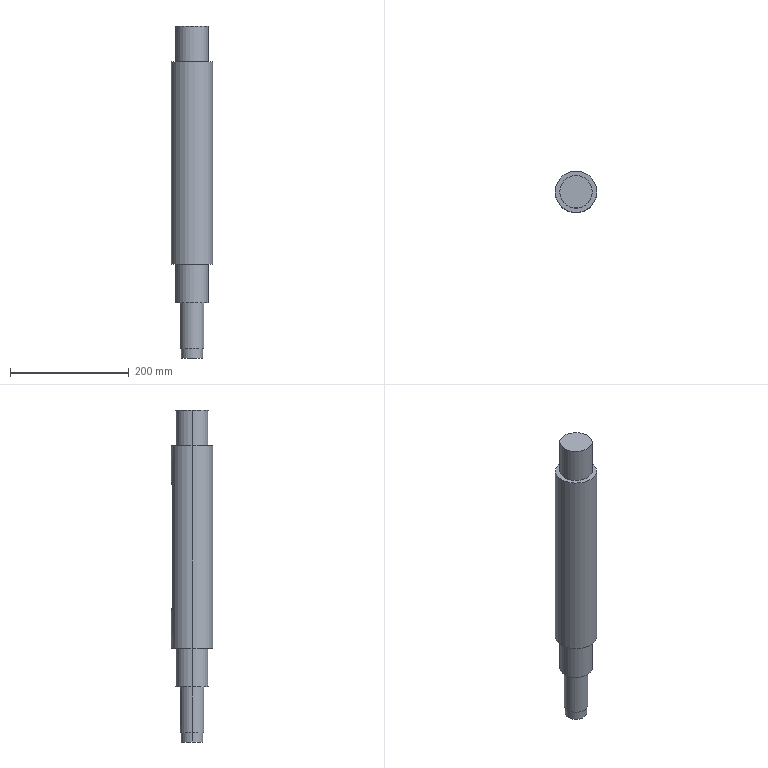Component | SolidWorks | Spindle-1 | 1 solid | 26 faces | box 70 x 70 x 560 mm | volume 1692469 mm3 | cylinder 14 | plane 12 | commonest cylinder face diameters 55 x4 70 x2 40 x2 36 x2 20 x2 12 x2
STEP:
#1=COLOUR_RGB('',0.7922,0.8196,0.9333);
#2=FILL_AREA_STYLE_COLOUR('',#1);
#3=FILL_AREA_STYLE('',(#2));
#4=SURFACE_STYLE_FILL_AREA(#3);
#5=SURFACE_SIDE_STYLE('',(#4));
#6=SURFACE_STYLE_USAGE(.BOTH.,#5);
#7=PRESENTATION_STYLE_ASSIGNMENT((#6));
#8=CARTESIAN_POINT('',(8.661,10.159,-3.886));
#9=VERTEX_POINT('',#8);
#10=CARTESIAN_POINT('',(8.661,10.159,3.988));
#11=VERTEX_POINT('',#10);
#12=CARTESIAN_POINT('',(8.661,10.159,9.106));
#13=DIRECTION('',(0.,0.,1.));
#14=VECTOR('',#13,39.37);
#15=LINE('',#12,#14);
#16=EDGE_CURVE('',#9,#11,#15,.T.);
#17=ORIENTED_EDGE('',*,*,#16,.T.);
#18=CARTESIAN_POINT('',(7.874,10.159,3.988));
#19=VERTEX_POINT('',#18);
#20=CARTESIAN_POINT('',(8.661,10.159,3.988));
#21=CARTESIAN_POINT('',(8.661,10.159,4.014));
#22=CARTESIAN_POINT('',(8.659,10.16,4.04));
#23=CARTESIAN_POINT('',(8.651,10.162,4.078));
#24=CARTESIAN_POINT('',(8.648,10.163,4.09));
#25=CARTESIAN_POINT('',(8.641,10.165,4.115));
#26=CARTESIAN_POINT('',(8.636,10.166,4.127));
#27=CARTESIAN_POINT('',(8.621,10.17,4.163));
#28=CARTESIAN_POINT('',(8.609,10.174,4.186));
#29=CARTESIAN_POINT('',(8.588,10.179,4.218));
#30=CARTESIAN_POINT('',(8.58,10.181,4.228));
#31=CARTESIAN_POINT('',(8.564,10.184,4.248));
#32=CARTESIAN_POINT('',(8.555,10.186,4.258));
#33=CARTESIAN_POINT('',(8.528,10.192,4.285));
#34=CARTESIAN_POINT('',(8.508,10.196,4.301));
#35=CARTESIAN_POINT('',(8.465,10.202,4.33));
#36=CARTESIAN_POINT('',(8.443,10.206,4.342));
#37=CARTESIAN_POINT('',(8.407,10.21,4.357));
#38=CARTESIAN_POINT('',(8.395,10.211,4.361));
#39=CARTESIAN_POINT('',(8.37,10.213,4.368));
#40=CARTESIAN_POINT('',(8.358,10.214,4.372));
#41=CARTESIAN_POINT('',(8.32,10.216,4.379));
#42=CARTESIAN_POINT('',(8.294,10.217,4.382));
#43=CARTESIAN_POINT('',(8.242,10.217,4.382));
#44=CARTESIAN_POINT('',(8.216,10.216,4.379));
#45=CARTESIAN_POINT('',(8.165,10.213,4.369));
#46=CARTESIAN_POINT('',(8.141,10.211,4.362));
#47=CARTESIAN_POINT('',(8.105,10.207,4.347));
#48=CARTESIAN_POINT('',(8.093,10.205,4.341));
#49=CARTESIAN_POINT('',(8.07,10.202,4.329));
#50=CARTESIAN_POINT('',(8.06,10.201,4.323));
#51=CARTESIAN_POINT('',(8.038,10.197,4.308));
#52=CARTESIAN_POINT('',(8.028,10.196,4.301));
#53=CARTESIAN_POINT('',(8.008,10.192,4.284));
#54=CARTESIAN_POINT('',(7.999,10.19,4.276));
#55=CARTESIAN_POINT('',(7.971,10.184,4.248));
#56=CARTESIAN_POINT('',(7.955,10.181,4.229));
#57=CARTESIAN_POINT('',(7.927,10.174,4.186));
#58=CARTESIAN_POINT('',(7.914,10.17,4.163));
#59=CARTESIAN_POINT('',(7.894,10.165,4.116));
#60=CARTESIAN_POINT('',(7.887,10.163,4.091));
#61=CARTESIAN_POINT('',(7.879,10.161,4.053));
#62=CARTESIAN_POINT('',(7.877,10.16,4.04));
#63=CARTESIAN_POINT('',(7.875,10.159,4.014));
#64=CARTESIAN_POINT('',(7.874,10.159,4.001));
#65=CARTESIAN_POINT('',(7.874,10.159,3.988));
#66=B_SPLINE_CURVE_WITH_KNOTS('',3,(#20,#21,#22,#23,#24,#25,#26,#27,#28,#29,#30,#31,#32,#33,#34,#35,#36,#37,#38,#39,#40,#41,#42,#43,#44,#45,#46,#47,#48,#49,#50,#51,#52,#53,#54,#55,#56,#57,#58,#59,#60,#61,#62,#63,#64,#65),.UNSPECIFIED.,.F.,.F.,(4,2,2,2,2,2,2,2,2,2,2,2,2,2,2,2,2,2,2,2,2,2,4),(0.,0.001964,0.002945,0.003927,0.005891,0.006873,0.007855,0.009818,0.01178,0.01276,0.01375,0.01571,0.01767,0.01964,0.02062,0.0216,0.02258,0.02356,0.02553,0.02749,0.02945,0.03044,0.03142),.UNSPECIFIED.);
#67=EDGE_CURVE('',#11,#19,#66,.T.);
#68=ORIENTED_EDGE('',*,*,#67,.T.);
#69=CARTESIAN_POINT('',(7.874,10.159,-3.886));
#70=VERTEX_POINT('',#69);
#71=CARTESIAN_POINT('',(7.874,10.159,9.106));
#72=DIRECTION('',(0.,0.,-1.));
#73=VECTOR('',#72,39.37);
#74=LINE('',#71,#73);
#75=EDGE_CURVE('',#19,#70,#74,.T.);
#76=ORIENTED_EDGE('',*,*,#75,.T.);
#77=CARTESIAN_POINT('',(7.874,10.159,-3.886));
#78=CARTESIAN_POINT('',(7.874,10.159,-3.912));
#79=CARTESIAN_POINT('',(7.877,10.16,-3.938));
#80=CARTESIAN_POINT('',(7.884,10.162,-3.976));
#81=CARTESIAN_POINT('',(7.887,10.163,-3.988));
#82=CARTESIAN_POINT('',(7.895,10.165,-4.013));
#83=CARTESIAN_POINT('',(7.899,10.166,-4.025));
#84=CARTESIAN_POINT('',(7.914,10.17,-4.061));
#85=CARTESIAN_POINT('',(7.926,10.174,-4.083));
#86=CARTESIAN_POINT('',(7.948,10.179,-4.115));
#87=CARTESIAN_POINT('',(7.955,10.181,-4.126));
#88=CARTESIAN_POINT('',(7.972,10.184,-4.146));
#89=CARTESIAN_POINT('',(7.98,10.186,-4.155));
#90=CARTESIAN_POINT('',(8.007,10.192,-4.182));
#91=CARTESIAN_POINT('',(8.027,10.196,-4.199));
#92=CARTESIAN_POINT('',(8.07,10.202,-4.227));
#93=CARTESIAN_POINT('',(8.093,10.206,-4.239));
#94=CARTESIAN_POINT('',(8.128,10.21,-4.254));
#95=CARTESIAN_POINT('',(8.14,10.211,-4.259));
#96=CARTESIAN_POINT('',(8.165,10.213,-4.266));
#97=CARTESIAN_POINT('',(8.178,10.214,-4.269));
#98=CARTESIAN_POINT('',(8.216,10.216,-4.277));
#99=CARTESIAN_POINT('',(8.242,10.217,-4.28));
#100=CARTESIAN_POINT('',(8.293,10.217,-4.28));
#101=CARTESIAN_POINT('',(8.319,10.216,-4.277));
#102=CARTESIAN_POINT('',(8.37,10.213,-4.267));
#103=CARTESIAN_POINT('',(8.395,10.211,-4.259));
#104=CARTESIAN_POINT('',(8.43,10.207,-4.245));
#105=CARTESIAN_POINT('',(8.442,10.205,-4.239));
#106=CARTESIAN_POINT('',(8.465,10.202,-4.227));
#107=CARTESIAN_POINT('',(8.476,10.201,-4.22));
#108=CARTESIAN_POINT('',(8.497,10.197,-4.206));
#109=CARTESIAN_POINT('',(8.507,10.196,-4.198));
#110=CARTESIAN_POINT('',(8.527,10.192,-4.182));
#111=CARTESIAN_POINT('',(8.537,10.19,-4.173));
#112=CARTESIAN_POINT('',(8.564,10.184,-4.146));
#113=CARTESIAN_POINT('',(8.58,10.181,-4.126));
#114=CARTESIAN_POINT('',(8.609,10.174,-4.084));
#115=CARTESIAN_POINT('',(8.621,10.17,-4.061));
#116=CARTESIAN_POINT('',(8.641,10.165,-4.013));
#117=CARTESIAN_POINT('',(8.649,10.163,-3.989));
#118=CARTESIAN_POINT('',(8.656,10.161,-3.951));
#119=CARTESIAN_POINT('',(8.658,10.16,-3.938));
#120=CARTESIAN_POINT('',(8.661,10.159,-3.912));
#121=CARTESIAN_POINT('',(8.661,10.159,-3.899));
#122=CARTESIAN_POINT('',(8.661,10.159,-3.886));
#123=B_SPLINE_CURVE_WITH_KNOTS('',3,(#77,#78,#79,#80,#81,#82,#83,#84,#85,#86,#87,#88,#89,#90,#91,#92,#93,#94,#95,#96,#97,#98,#99,#100,#101,#102,#103,#104,#105,#106,#107,#108,#109,#110,#111,#112,#113,#114,#115,#116,#117,#118,#119,#120,#121,#122),.UNSPECIFIED.,.F.,.F.,(4,2,2,2,2,2,2,2,2,2,2,2,2,2,2,2,2,2,2,2,2,2,4),(0.,0.001964,0.002945,0.003927,0.005891,0.006873,0.007855,0.009818,0.01178,0.01276,0.01375,0.01571,0.01767,0.01964,0.02062,0.0216,0.02258,0.02356,0.02553,0.02749,0.02945,0.03044,0.03142),.UNSPECIFIED.);
#124=EDGE_CURVE('',#70,#9,#123,.T.);
#125=ORIENTED_EDGE('',*,*,#124,.T.);
#126=EDGE_LOOP('',(#17,#68,#76,#125));
#127=FACE_BOUND('',#126,.T.);
#128=CARTESIAN_POINT('',(9.646,8.839,-6.72));
#129=VERTEX_POINT('',#128);
#130=CARTESIAN_POINT('',(6.89,8.839,-6.72));
#131=VERTEX_POINT('',#130);
#132=CARTESIAN_POINT('',(8.268,8.839,-6.72));
#133=DIRECTION('',(0.,0.,1.));
#134=DIRECTION('',(1.,0.,0.));
#135=AXIS2_PLACEMENT_3D('',#132,#133,#134);
#136=CIRCLE('',#135,1.378);
#137=EDGE_CURVE('',#129,#131,#136,.T.);
#138=ORIENTED_EDGE('',*,*,#137,.T.);
#139=CARTESIAN_POINT('',(6.89,8.839,6.744));
#140=VERTEX_POINT('',#139);
#141=CARTESIAN_POINT('',(6.89,8.839,9.106));
#142=DIRECTION('',(0.,0.,1.));
#143=VECTOR('',#142,39.37);
#144=LINE('',#141,#143);
#145=EDGE_CURVE('',#131,#140,#144,.T.);
#146=ORIENTED_EDGE('',*,*,#145,.T.);
#147=CARTESIAN_POINT('',(9.646,8.839,6.744));
#148=VERTEX_POINT('',#147);
#149=CARTESIAN_POINT('',(8.268,8.839,6.744));
#150=DIRECTION('',(0.,0.,-1.));
#151=DIRECTION('',(1.,0.,0.));
#152=AXIS2_PLACEMENT_3D('',#149,#150,#151);
#153=CIRCLE('',#152,1.378);
#154=EDGE_CURVE('',#140,#148,#153,.T.);
#155=ORIENTED_EDGE('',*,*,#154,.T.);
#156=CARTESIAN_POINT('',(9.646,8.839,9.106));
#157=DIRECTION('',(0.,0.,1.));
#158=VECTOR('',#157,39.37);
#159=LINE('',#156,#158);
#160=EDGE_CURVE('',#129,#148,#159,.T.);
#161=ORIENTED_EDGE('',*,*,#160,.F.);
#162=EDGE_LOOP('',(#138,#146,#155,#161));
#163=FACE_OUTER_BOUND('',#162,.T.);
#164=CARTESIAN_POINT('',(8.268,8.839,9.106));
#165=DIRECTION('',(0.,0.,1.));
#166=DIRECTION('',(1.,0.,0.));
#167=AXIS2_PLACEMENT_3D('',#164,#165,#166);
#168=CYLINDRICAL_SURFACE('',#167,1.378);
#169=ADVANCED_FACE('',(#127,#163),#168,.T.);
#170=CARTESIAN_POINT('',(9.35,8.839,6.744));
#171=VERTEX_POINT('',#170);
#172=CARTESIAN_POINT('',(7.185,8.839,6.744));
#173=VERTEX_POINT('',#172);
#174=CARTESIAN_POINT('',(8.268,8.839,6.744));
#175=DIRECTION('',(0.,0.,1.));
#176=DIRECTION('',(1.,0.,0.));
#177=AXIS2_PLACEMENT_3D('',#174,#175,#176);
#178=CIRCLE('',#177,1.083);
#179=EDGE_CURVE('',#171,#173,#178,.T.);
#180=ORIENTED_EDGE('',*,*,#179,.T.);
#181=CARTESIAN_POINT('',(7.185,8.839,9.106));
#182=VERTEX_POINT('',#181);
#183=CARTESIAN_POINT('',(7.185,8.839,9.106));
#184=DIRECTION('',(0.,0.,1.));
#185=VECTOR('',#184,39.37);
#186=LINE('',#183,#185);
#187=EDGE_CURVE('',#173,#182,#186,.T.);
#188=ORIENTED_EDGE('',*,*,#187,.T.);
#189=CARTESIAN_POINT('',(9.35,8.839,9.106));
#190=VERTEX_POINT('',#189);
#191=CARTESIAN_POINT('',(8.268,8.839,9.106));
#192=DIRECTION('',(0.,0.,-1.));
#193=DIRECTION('',(1.,0.,0.));
#194=AXIS2_PLACEMENT_3D('',#191,#192,#193);
#195=CIRCLE('',#194,1.083);
#196=EDGE_CURVE('',#182,#190,#195,.T.);
#197=ORIENTED_EDGE('',*,*,#196,.T.);
#198=CARTESIAN_POINT('',(9.35,8.839,9.106));
#199=DIRECTION('',(0.,0.,1.));
#200=VECTOR('',#199,39.37);
#201=LINE('',#198,#200);
#202=EDGE_CURVE('',#171,#190,#201,.T.);
#203=ORIENTED_EDGE('',*,*,#202,.F.);
#204=EDGE_LOOP('',(#180,#188,#197,#203));
#205=FACE_OUTER_BOUND('',#204,.T.);
#206=CARTESIAN_POINT('',(8.268,8.839,9.106));
#207=DIRECTION('',(0.,0.,1.));
#208=DIRECTION('',(1.,0.,0.));
#209=AXIS2_PLACEMENT_3D('',#206,#207,#208);
#210=CYLINDRICAL_SURFACE('',#209,1.083);
#211=ADVANCED_FACE('',(#205),#210,.T.);
#212=CARTESIAN_POINT('',(9.35,8.839,-9.28));
#213=VERTEX_POINT('',#212);
#214=CARTESIAN_POINT('',(7.185,8.839,-9.28));
#215=VERTEX_POINT('',#214);
#216=CARTESIAN_POINT('',(8.268,8.839,-9.28));
#217=DIRECTION('',(0.,0.,1.));
#218=DIRECTION('',(1.,0.,0.));
#219=AXIS2_PLACEMENT_3D('',#216,#217,#218);
#220=CIRCLE('',#219,1.083);
#221=EDGE_CURVE('',#213,#215,#220,.T.);
#222=ORIENTED_EDGE('',*,*,#221,.T.);
#223=CARTESIAN_POINT('',(7.185,8.839,-6.72));
#224=VERTEX_POINT('',#223);
#225=CARTESIAN_POINT('',(7.185,8.839,9.106));
#226=DIRECTION('',(0.,0.,1.));
#227=VECTOR('',#226,39.37);
#228=LINE('',#225,#227);
#229=EDGE_CURVE('',#215,#224,#228,.T.);
#230=ORIENTED_EDGE('',*,*,#229,.T.);
#231=CARTESIAN_POINT('',(9.35,8.839,-6.72));
#232=VERTEX_POINT('',#231);
#233=CARTESIAN_POINT('',(8.268,8.839,-6.72));
#234=DIRECTION('',(0.,0.,-1.));
#235=DIRECTION('',(1.,0.,0.));
#236=AXIS2_PLACEMENT_3D('',#233,#234,#235);
#237=CIRCLE('',#236,1.083);
#238=EDGE_CURVE('',#224,#232,#237,.T.);
#239=ORIENTED_EDGE('',*,*,#238,.T.);
#240=CARTESIAN_POINT('',(9.35,8.839,9.106));
#241=DIRECTION('',(0.,0.,1.));
#242=VECTOR('',#241,39.37);
#243=LINE('',#240,#242);
#244=EDGE_CURVE('',#213,#232,#243,.T.);
#245=ORIENTED_EDGE('',*,*,#244,.F.);
#246=EDGE_LOOP('',(#222,#230,#239,#245));
#247=FACE_OUTER_BOUND('',#246,.T.);
#248=CARTESIAN_POINT('',(8.268,8.839,9.106));
#249=DIRECTION('',(0.,0.,1.));
#250=DIRECTION('',(1.,0.,0.));
#251=AXIS2_PLACEMENT_3D('',#248,#249,#250);
#252=CYLINDRICAL_SURFACE('',#251,1.083);
#253=ADVANCED_FACE('',(#247),#252,.T.);
#254=CARTESIAN_POINT('',(8.504,9.59,-11.72));
#255=VERTEX_POINT('',#254);
#256=CARTESIAN_POINT('',(8.504,9.59,-9.713));
#257=VERTEX_POINT('',#256);
#258=CARTESIAN_POINT('',(8.504,9.59,9.106));
#259=DIRECTION('',(0.,0.,1.));
#260=VECTOR('',#259,39.37);
#261=LINE('',#258,#260);
#262=EDGE_CURVE('',#255,#257,#261,.T.);
#263=ORIENTED_EDGE('',*,*,#262,.T.);
#264=CARTESIAN_POINT('',(8.031,9.59,-9.713));
#265=VERTEX_POINT('',#264);
#266=CARTESIAN_POINT('',(8.504,9.59,-9.713));
#267=CARTESIAN_POINT('',(8.504,9.59,-9.697));
#268=CARTESIAN_POINT('',(8.502,9.59,-9.681));
#269=CARTESIAN_POINT('',(8.498,9.592,-9.659));
#270=CARTESIAN_POINT('',(8.496,9.592,-9.651));
#271=CARTESIAN_POINT('',(8.491,9.594,-9.636));
#272=CARTESIAN_POINT('',(8.489,9.594,-9.629));
#273=CARTESIAN_POINT('',(8.48,9.597,-9.608));
#274=CARTESIAN_POINT('',(8.473,9.599,-9.594));
#275=CARTESIAN_POINT('',(8.46,9.602,-9.575));
#276=CARTESIAN_POINT('',(8.455,9.603,-9.569));
#277=CARTESIAN_POINT('',(8.445,9.606,-9.557));
#278=CARTESIAN_POINT('',(8.44,9.607,-9.551));
#279=CARTESIAN_POINT('',(8.424,9.61,-9.535));
#280=CARTESIAN_POINT('',(8.412,9.613,-9.525));
#281=CARTESIAN_POINT('',(8.386,9.617,-9.508));
#282=CARTESIAN_POINT('',(8.373,9.619,-9.5));
#283=CARTESIAN_POINT('',(8.351,9.622,-9.492));
#284=CARTESIAN_POINT('',(8.344,9.622,-9.489));
#285=CARTESIAN_POINT('',(8.329,9.624,-9.484));
#286=CARTESIAN_POINT('',(8.322,9.624,-9.483));
#287=CARTESIAN_POINT('',(8.299,9.626,-9.478));
#288=CARTESIAN_POINT('',(8.283,9.626,-9.476));
#289=CARTESIAN_POINT('',(8.252,9.626,-9.476));
#290=CARTESIAN_POINT('',(8.237,9.626,-9.478));
#291=CARTESIAN_POINT('',(8.206,9.624,-9.484));
#292=CARTESIAN_POINT('',(8.192,9.622,-9.488));
#293=CARTESIAN_POINT('',(8.17,9.62,-9.497));
#294=CARTESIAN_POINT('',(8.163,9.619,-9.501));
#295=CARTESIAN_POINT('',(8.149,9.617,-9.508));
#296=CARTESIAN_POINT('',(8.143,9.616,-9.512));
#297=CARTESIAN_POINT('',(8.13,9.614,-9.521));
#298=CARTESIAN_POINT('',(8.124,9.613,-9.525));
#299=CARTESIAN_POINT('',(8.112,9.61,-9.535));
#300=CARTESIAN_POINT('',(8.106,9.609,-9.54));
#301=CARTESIAN_POINT('',(8.09,9.606,-9.556));
#302=CARTESIAN_POINT('',(8.08,9.603,-9.568));
#303=CARTESIAN_POINT('',(8.063,9.599,-9.594));
#304=CARTESIAN_POINT('',(8.056,9.597,-9.608));
#305=CARTESIAN_POINT('',(8.044,9.593,-9.636));
#306=CARTESIAN_POINT('',(8.039,9.592,-9.651));
#307=CARTESIAN_POINT('',(8.033,9.59,-9.681));
#308=CARTESIAN_POINT('',(8.031,9.59,-9.697));
#309=CARTESIAN_POINT('',(8.031,9.59,-9.713));
#310=B_SPLINE_CURVE_WITH_KNOTS('',3,(#266,#267,#268,#269,#270,#271,#272,#273,#274,#275,#276,#277,#278,#279,#280,#281,#282,#283,#284,#285,#286,#287,#288,#289,#290,#291,#292,#293,#294,#295,#296,#297,#298,#299,#300,#301,#302,#303,#304,#305,#306,#307,#308,#309),.UNSPECIFIED.,.F.,.F.,(4,2,2,2,2,2,2,2,2,2,2,2,2,2,2,2,2,2,2,2,2,4),(0.,0.001179,0.001768,0.002358,0.003536,0.004126,0.004715,0.005894,0.007073,0.007662,0.008252,0.009431,0.01061,0.01179,0.01238,0.01297,0.01356,0.01415,0.01532,0.0165,0.01768,0.01886),.UNSPECIFIED.);
#311=EDGE_CURVE('',#257,#265,#310,.T.);
#312=ORIENTED_EDGE('',*,*,#311,.T.);
#313=CARTESIAN_POINT('',(8.031,9.59,-11.72));
#314=VERTEX_POINT('',#313);
#315=CARTESIAN_POINT('',(8.031,9.59,9.106));
#316=DIRECTION('',(0.,0.,-1.));
#317=VECTOR('',#316,39.37);
#318=LINE('',#315,#317);
#319=EDGE_CURVE('',#265,#314,#318,.T.);
#320=ORIENTED_EDGE('',*,*,#319,.T.);
#321=CARTESIAN_POINT('',(8.031,9.59,-11.72));
#322=CARTESIAN_POINT('',(8.031,9.59,-11.736));
#323=CARTESIAN_POINT('',(8.033,9.59,-11.752));
#324=CARTESIAN_POINT('',(8.038,9.592,-11.774));
#325=CARTESIAN_POINT('',(8.039,9.592,-11.782));
#326=CARTESIAN_POINT('',(8.044,9.594,-11.797));
#327=CARTESIAN_POINT('',(8.047,9.594,-11.804));
#328=CARTESIAN_POINT('',(8.056,9.597,-11.825));
#329=CARTESIAN_POINT('',(8.063,9.599,-11.839));
#330=CARTESIAN_POINT('',(8.076,9.602,-11.858));
#331=CARTESIAN_POINT('',(8.08,9.603,-11.864));
#332=CARTESIAN_POINT('',(8.09,9.606,-11.876));
#333=CARTESIAN_POINT('',(8.095,9.607,-11.882));
#334=CARTESIAN_POINT('',(8.111,9.61,-11.898));
#335=CARTESIAN_POINT('',(8.123,9.613,-11.908));
#336=CARTESIAN_POINT('',(8.149,9.617,-11.925));
#337=CARTESIAN_POINT('',(8.163,9.619,-11.933));
#338=CARTESIAN_POINT('',(8.184,9.622,-11.941));
#339=CARTESIAN_POINT('',(8.191,9.622,-11.944));
#340=CARTESIAN_POINT('',(8.206,9.624,-11.949));
#341=CARTESIAN_POINT('',(8.214,9.624,-11.951));
#342=CARTESIAN_POINT('',(8.237,9.626,-11.955));
#343=CARTESIAN_POINT('',(8.252,9.626,-11.957));
#344=CARTESIAN_POINT('',(8.283,9.626,-11.957));
#345=CARTESIAN_POINT('',(8.299,9.626,-11.955));
#346=CARTESIAN_POINT('',(8.329,9.624,-11.949));
#347=CARTESIAN_POINT('',(8.344,9.622,-11.945));
#348=CARTESIAN_POINT('',(8.365,9.62,-11.936));
#349=CARTESIAN_POINT('',(8.372,9.619,-11.932));
#350=CARTESIAN_POINT('',(8.386,9.617,-11.925));
#351=CARTESIAN_POINT('',(8.393,9.616,-11.921));
#352=CARTESIAN_POINT('',(8.405,9.614,-11.913));
#353=CARTESIAN_POINT('',(8.412,9.613,-11.908));
#354=CARTESIAN_POINT('',(8.423,9.61,-11.898));
#355=CARTESIAN_POINT('',(8.429,9.609,-11.893));
#356=CARTESIAN_POINT('',(8.446,9.606,-11.877));
#357=CARTESIAN_POINT('',(8.455,9.603,-11.865));
#358=CARTESIAN_POINT('',(8.472,9.599,-11.839));
#359=CARTESIAN_POINT('',(8.48,9.597,-11.826));
#360=CARTESIAN_POINT('',(8.492,9.593,-11.797));
#361=CARTESIAN_POINT('',(8.496,9.592,-11.782));
#362=CARTESIAN_POINT('',(8.502,9.59,-11.752));
#363=CARTESIAN_POINT('',(8.504,9.59,-11.736));
#364=CARTESIAN_POINT('',(8.504,9.59,-11.72));
#365=B_SPLINE_CURVE_WITH_KNOTS('',3,(#321,#322,#323,#324,#325,#326,#327,#328,#329,#330,#331,#332,#333,#334,#335,#336,#337,#338,#339,#340,#341,#342,#343,#344,#345,#346,#347,#348,#349,#350,#351,#352,#353,#354,#355,#356,#357,#358,#359,#360,#361,#362,#363,#364),.UNSPECIFIED.,.F.,.F.,(4,2,2,2,2,2,2,2,2,2,2,2,2,2,2,2,2,2,2,2,2,4),(0.,0.001179,0.001768,0.002358,0.003536,0.004126,0.004715,0.005894,0.007073,0.007662,0.008252,0.009431,0.01061,0.01179,0.01238,0.01297,0.01356,0.01415,0.01532,0.0165,0.01768,0.01886),.UNSPECIFIED.);
#366=EDGE_CURVE('',#314,#255,#365,.T.);
#367=ORIENTED_EDGE('',*,*,#366,.T.);
#368=EDGE_LOOP('',(#263,#312,#320,#367));
#369=FACE_BOUND('',#368,.T.);
#370=CARTESIAN_POINT('',(9.055,8.839,-12.311));
#371=VERTEX_POINT('',#370);
#372=CARTESIAN_POINT('',(7.48,8.839,-12.311));
#373=VERTEX_POINT('',#372);
#374=CARTESIAN_POINT('',(8.268,8.839,-12.311));
#375=DIRECTION('',(0.,0.,1.));
#376=DIRECTION('',(1.,0.,0.));
#377=AXIS2_PLACEMENT_3D('',#374,#375,#376);
#378=CIRCLE('',#377,0.7874);
#379=EDGE_CURVE('',#371,#373,#378,.T.);
#380=ORIENTED_EDGE('',*,*,#379,.T.);
#381=CARTESIAN_POINT('',(7.48,8.839,-9.28));
#382=VERTEX_POINT('',#381);
#383=CARTESIAN_POINT('',(7.48,8.839,9.106));
#384=DIRECTION('',(0.,0.,1.));
#385=VECTOR('',#384,39.37);
#386=LINE('',#383,#385);
#387=EDGE_CURVE('',#373,#382,#386,.T.);
#388=ORIENTED_EDGE('',*,*,#387,.T.);
#389=CARTESIAN_POINT('',(9.055,8.839,-9.28));
#390=VERTEX_POINT('',#389);
#391=CARTESIAN_POINT('',(8.268,8.839,-9.28));
#392=DIRECTION('',(0.,0.,-1.));
#393=DIRECTION('',(1.,0.,0.));
#394=AXIS2_PLACEMENT_3D('',#391,#392,#393);
#395=CIRCLE('',#394,0.7874);
#396=EDGE_CURVE('',#382,#390,#395,.T.);
#397=ORIENTED_EDGE('',*,*,#396,.T.);
#398=CARTESIAN_POINT('',(9.055,8.839,9.106));
#399=DIRECTION('',(0.,0.,1.));
#400=VECTOR('',#399,39.37);
#401=LINE('',#398,#400);
#402=EDGE_CURVE('',#371,#390,#401,.T.);
#403=ORIENTED_EDGE('',*,*,#402,.F.);
#404=EDGE_LOOP('',(#380,#388,#397,#403));
#405=FACE_OUTER_BOUND('',#404,.T.);
#406=CARTESIAN_POINT('',(8.268,8.839,9.106));
#407=DIRECTION('',(0.,0.,1.));
#408=DIRECTION('',(1.,0.,0.));
#409=AXIS2_PLACEMENT_3D('',#406,#407,#408);
#410=CYLINDRICAL_SURFACE('',#409,0.7874);
#411=ADVANCED_FACE('',(#369,#405),#410,.T.);
#412=CARTESIAN_POINT('',(8.976,8.839,-12.941));
#413=VERTEX_POINT('',#412);
#414=CARTESIAN_POINT('',(7.559,8.839,-12.941));
#415=VERTEX_POINT('',#414);
#416=CARTESIAN_POINT('',(8.268,8.839,-12.941));
#417=DIRECTION('',(0.,0.,1.));
#418=DIRECTION('',(1.,0.,0.));
#419=AXIS2_PLACEMENT_3D('',#416,#417,#418);
#420=CIRCLE('',#419,0.7087);
#421=EDGE_CURVE('',#413,#415,#420,.T.);
#422=ORIENTED_EDGE('',*,*,#421,.T.);
#423=CARTESIAN_POINT('',(7.559,8.839,-12.311));
#424=VERTEX_POINT('',#423);
#425=CARTESIAN_POINT('',(7.559,8.839,9.106));
#426=DIRECTION('',(0.,0.,1.));
#427=VECTOR('',#426,39.37);
#428=LINE('',#425,#427);
#429=EDGE_CURVE('',#415,#424,#428,.T.);
#430=ORIENTED_EDGE('',*,*,#429,.T.);
#431=CARTESIAN_POINT('',(8.976,8.839,-12.311));
#432=VERTEX_POINT('',#431);
#433=CARTESIAN_POINT('',(8.268,8.839,-12.311));
#434=DIRECTION('',(0.,0.,-1.));
#435=DIRECTION('',(1.,0.,0.));
#436=AXIS2_PLACEMENT_3D('',#433,#434,#435);
#437=CIRCLE('',#436,0.7087);
#438=EDGE_CURVE('',#424,#432,#437,.T.);
#439=ORIENTED_EDGE('',*,*,#438,.T.);
#440=CARTESIAN_POINT('',(8.976,8.839,9.106));
#441=DIRECTION('',(0.,0.,1.));
#442=VECTOR('',#441,39.37);
#443=LINE('',#440,#442);
#444=EDGE_CURVE('',#413,#432,#443,.T.);
#445=ORIENTED_EDGE('',*,*,#444,.F.);
#446=EDGE_LOOP('',(#422,#430,#439,#445));
#447=FACE_OUTER_BOUND('',#446,.T.);
#448=CARTESIAN_POINT('',(8.268,8.839,9.106));
#449=DIRECTION('',(0.,0.,1.));
#450=DIRECTION('',(1.,0.,0.));
#451=AXIS2_PLACEMENT_3D('',#448,#449,#450);
#452=CYLINDRICAL_SURFACE('',#451,0.7087);
#453=ADVANCED_FACE('',(#447),#452,.T.);
#454=ORIENTED_EDGE('',*,*,#145,.F.);
#455=CARTESIAN_POINT('',(8.268,8.839,-6.72));
#456=DIRECTION('',(0.,0.,1.));
#457=DIRECTION('',(1.,0.,0.));
#458=AXIS2_PLACEMENT_3D('',#455,#456,#457);
#459=CIRCLE('',#458,1.378);
#460=EDGE_CURVE('',#131,#129,#459,.T.);
#461=ORIENTED_EDGE('',*,*,#460,.T.);
#462=ORIENTED_EDGE('',*,*,#160,.T.);
#463=CARTESIAN_POINT('',(8.268,8.839,6.744));
#464=DIRECTION('',(0.,0.,-1.));
#465=DIRECTION('',(1.,0.,0.));
#466=AXIS2_PLACEMENT_3D('',#463,#464,#465);
#467=CIRCLE('',#466,1.378);
#468=EDGE_CURVE('',#148,#140,#467,.T.);
#469=ORIENTED_EDGE('',*,*,#468,.T.);
#470=EDGE_LOOP('',(#454,#461,#462,#469));
#471=FACE_OUTER_BOUND('',#470,.T.);
#472=CARTESIAN_POINT('',(8.268,8.839,9.106));
#473=DIRECTION('',(0.,0.,1.));
#474=DIRECTION('',(1.,0.,0.));
#475=AXIS2_PLACEMENT_3D('',#472,#473,#474);
#476=CYLINDRICAL_SURFACE('',#475,1.378);
#477=ADVANCED_FACE('',(#471),#476,.T.);
#478=ORIENTED_EDGE('',*,*,#468,.F.);
#479=ORIENTED_EDGE('',*,*,#154,.F.);
#480=EDGE_LOOP('',(#478,#479));
#481=FACE_OUTER_BOUND('',#480,.T.);
#482=ORIENTED_EDGE('',*,*,#179,.F.);
#483=CARTESIAN_POINT('',(8.268,8.839,6.744));
#484=DIRECTION('',(0.,0.,1.));
#485=DIRECTION('',(1.,0.,0.));
#486=AXIS2_PLACEMENT_3D('',#483,#484,#485);
#487=CIRCLE('',#486,1.083);
#488=EDGE_CURVE('',#173,#171,#487,.T.);
#489=ORIENTED_EDGE('',*,*,#488,.F.);
#490=EDGE_LOOP('',(#482,#489));
#491=FACE_BOUND('',#490,.T.);
#492=CARTESIAN_POINT('',(8.268,9.921,6.744));
#493=DIRECTION('',(0.,0.,-1.));
#494=DIRECTION('',(-1.,0.,0.));
#495=AXIS2_PLACEMENT_3D('',#492,#493,#494);
#496=PLANE('',#495);
#497=ADVANCED_FACE('',(#481,#491),#496,.F.);
#498=CARTESIAN_POINT('',(8.268,8.839,-6.72));
#499=DIRECTION('',(0.,0.,-1.));
#500=DIRECTION('',(1.,0.,0.));
#501=AXIS2_PLACEMENT_3D('',#498,#499,#500);
#502=CIRCLE('',#501,1.083);
#503=EDGE_CURVE('',#232,#224,#502,.T.);
#504=ORIENTED_EDGE('',*,*,#503,.F.);
#505=ORIENTED_EDGE('',*,*,#238,.F.);
#506=EDGE_LOOP('',(#504,#505));
#507=FACE_BOUND('',#506,.T.);
#508=ORIENTED_EDGE('',*,*,#137,.F.);
#509=ORIENTED_EDGE('',*,*,#460,.F.);
#510=EDGE_LOOP('',(#508,#509));
#511=FACE_OUTER_BOUND('',#510,.T.);
#512=CARTESIAN_POINT('',(8.268,10.217,-6.72));
#513=DIRECTION('',(0.,0.,1.));
#514=DIRECTION('',(1.,0.,0.));
#515=AXIS2_PLACEMENT_3D('',#512,#513,#514);
#516=PLANE('',#515);
#517=ADVANCED_FACE('',(#507,#511),#516,.F.);
#518=ORIENTED_EDGE('',*,*,#187,.F.);
#519=ORIENTED_EDGE('',*,*,#488,.T.);
#520=ORIENTED_EDGE('',*,*,#202,.T.);
#521=CARTESIAN_POINT('',(8.268,8.839,9.106));
#522=DIRECTION('',(0.,0.,-1.));
#523=DIRECTION('',(1.,0.,0.));
#524=AXIS2_PLACEMENT_3D('',#521,#522,#523);
#525=CIRCLE('',#524,1.083);
#526=EDGE_CURVE('',#190,#182,#525,.T.);
#527=ORIENTED_EDGE('',*,*,#526,.T.);
#528=EDGE_LOOP('',(#518,#519,#520,#527));
#529=FACE_OUTER_BOUND('',#528,.T.);
#530=CARTESIAN_POINT('',(8.268,8.839,9.106));
#531=DIRECTION('',(0.,0.,1.));
#532=DIRECTION('',(1.,0.,0.));
#533=AXIS2_PLACEMENT_3D('',#530,#531,#532);
#534=CYLINDRICAL_SURFACE('',#533,1.083);
#535=ADVANCED_FACE('',(#529),#534,.T.);
#536=CARTESIAN_POINT('',(7.874,9.921,3.988));
#537=VERTEX_POINT('',#536);
#538=CARTESIAN_POINT('',(8.661,9.921,3.988));
#539=VERTEX_POINT('',#538);
#540=CARTESIAN_POINT('',(8.268,9.921,3.988));
#541=DIRECTION('',(0.,1.,0.));
#542=DIRECTION('',(1.,0.,0.));
#543=AXIS2_PLACEMENT_3D('',#540,#541,#542);
#544=CIRCLE('',#543,0.3937);
#545=EDGE_CURVE('',#537,#539,#544,.T.);
#546=ORIENTED_EDGE('',*,*,#545,.F.);
#547=CARTESIAN_POINT('',(7.874,9.921,3.988));
#548=DIRECTION('',(0.,-1.,0.));
#549=VECTOR('',#548,39.37);
#550=LINE('',#547,#549);
#551=EDGE_CURVE('',#19,#537,#550,.T.);
#552=ORIENTED_EDGE('',*,*,#551,.F.);
#553=ORIENTED_EDGE('',*,*,#67,.F.);
#554=CARTESIAN_POINT('',(8.661,9.921,3.988));
#555=DIRECTION('',(0.,1.,0.));
#556=VECTOR('',#555,39.37);
#557=LINE('',#554,#556);
#558=EDGE_CURVE('',#539,#11,#557,.T.);
#559=ORIENTED_EDGE('',*,*,#558,.F.);
#560=EDGE_LOOP('',(#546,#552,#553,#559));
#561=FACE_OUTER_BOUND('',#560,.T.);
#562=CARTESIAN_POINT('',(8.268,9.921,3.988));
#563=DIRECTION('',(0.,1.,0.));
#564=DIRECTION('',(1.,0.,0.));
#565=AXIS2_PLACEMENT_3D('',#562,#563,#564);
#566=CYLINDRICAL_SURFACE('',#565,0.3937);
#567=ADVANCED_FACE('',(#561),#566,.F.);
#568=CARTESIAN_POINT('',(8.661,9.921,-3.886));
#569=VERTEX_POINT('',#568);
#570=CARTESIAN_POINT('',(8.661,9.921,3.988));
#571=DIRECTION('',(0.,0.,-1.));
#572=VECTOR('',#571,39.37);
#573=LINE('',#570,#572);
#574=EDGE_CURVE('',#539,#569,#573,.T.);
#575=ORIENTED_EDGE('',*,*,#574,.F.);
#576=ORIENTED_EDGE('',*,*,#558,.T.);
#577=ORIENTED_EDGE('',*,*,#16,.F.);
#578=CARTESIAN_POINT('',(8.661,9.921,-3.886));
#579=DIRECTION('',(0.,1.,0.));
#580=VECTOR('',#579,39.37);
#581=LINE('',#578,#580);
#582=EDGE_CURVE('',#569,#9,#581,.T.);
#583=ORIENTED_EDGE('',*,*,#582,.F.);
#584=EDGE_LOOP('',(#575,#576,#577,#583));
#585=FACE_OUTER_BOUND('',#584,.T.);
#586=CARTESIAN_POINT('',(8.661,9.921,3.988));
#587=DIRECTION('',(1.,0.,0.));
#588=DIRECTION('',(0.,0.,-1.));
#589=AXIS2_PLACEMENT_3D('',#586,#587,#588);
#590=PLANE('',#589);
#591=ADVANCED_FACE('',(#585),#590,.F.);
#592=CARTESIAN_POINT('',(7.874,9.921,-3.886));
#593=VERTEX_POINT('',#592);
#594=CARTESIAN_POINT('',(8.268,9.921,-3.886));
#595=DIRECTION('',(0.,1.,0.));
#596=DIRECTION('',(1.,0.,0.));
#597=AXIS2_PLACEMENT_3D('',#594,#595,#596);
#598=CIRCLE('',#597,0.3937);
#599=EDGE_CURVE('',#569,#593,#598,.T.);
#600=ORIENTED_EDGE('',*,*,#599,.F.);
#601=ORIENTED_EDGE('',*,*,#582,.T.);
#602=ORIENTED_EDGE('',*,*,#124,.F.);
#603=CARTESIAN_POINT('',(7.874,9.921,-3.886));
#604=DIRECTION('',(0.,1.,0.));
#605=VECTOR('',#604,39.37);
#606=LINE('',#603,#605);
#607=EDGE_CURVE('',#593,#70,#606,.T.);
#608=ORIENTED_EDGE('',*,*,#607,.F.);
#609=EDGE_LOOP('',(#600,#601,#602,#608));
#610=FACE_OUTER_BOUND('',#609,.T.);
#611=CARTESIAN_POINT('',(8.268,9.921,-3.886));
#612=DIRECTION('',(0.,1.,0.));
#613=DIRECTION('',(1.,0.,0.));
#614=AXIS2_PLACEMENT_3D('',#611,#612,#613);
#615=CYLINDRICAL_SURFACE('',#614,0.3937);
#616=ADVANCED_FACE('',(#610),#615,.F.);
#617=CARTESIAN_POINT('',(7.874,9.921,3.988));
#618=DIRECTION('',(0.,0.,1.));
#619=VECTOR('',#618,39.37);
#620=LINE('',#617,#619);
#621=EDGE_CURVE('',#593,#537,#620,.T.);
#622=ORIENTED_EDGE('',*,*,#621,.F.);
#623=ORIENTED_EDGE('',*,*,#607,.T.);
#624=ORIENTED_EDGE('',*,*,#75,.F.);
#625=ORIENTED_EDGE('',*,*,#551,.T.);
#626=EDGE_LOOP('',(#622,#623,#624,#625));
#627=FACE_OUTER_BOUND('',#626,.T.);
#628=CARTESIAN_POINT('',(7.874,9.921,3.988));
#629=DIRECTION('',(-1.,0.,0.));
#630=DIRECTION('',(0.,0.,1.));
#631=AXIS2_PLACEMENT_3D('',#628,#629,#630);
#632=PLANE('',#631);
#633=ADVANCED_FACE('',(#627),#632,.F.);
#634=ORIENTED_EDGE('',*,*,#229,.F.);
#635=CARTESIAN_POINT('',(8.268,8.839,-9.28));
#636=DIRECTION('',(0.,0.,1.));
#637=DIRECTION('',(1.,0.,0.));
#638=AXIS2_PLACEMENT_3D('',#635,#636,#637);
#639=CIRCLE('',#638,1.083);
#640=EDGE_CURVE('',#215,#213,#639,.T.);
#641=ORIENTED_EDGE('',*,*,#640,.T.);
#642=ORIENTED_EDGE('',*,*,#244,.T.);
#643=ORIENTED_EDGE('',*,*,#503,.T.);
#644=EDGE_LOOP('',(#634,#641,#642,#643));
#645=FACE_OUTER_BOUND('',#644,.T.);
#646=CARTESIAN_POINT('',(8.268,8.839,9.106));
#647=DIRECTION('',(0.,0.,1.));
#648=DIRECTION('',(1.,0.,0.));
#649=AXIS2_PLACEMENT_3D('',#646,#647,#648);
#650=CYLINDRICAL_SURFACE('',#649,1.083);
#651=ADVANCED_FACE('',(#645),#650,.T.);
#652=ORIENTED_EDGE('',*,*,#526,.F.);
#653=ORIENTED_EDGE('',*,*,#196,.F.);
#654=EDGE_LOOP('',(#652,#653));
#655=FACE_OUTER_BOUND('',#654,.T.);
#656=CARTESIAN_POINT('',(8.268,8.839,9.106));
#657=DIRECTION('',(0.,0.,-1.));
#658=DIRECTION('',(-1.,0.,0.));
#659=AXIS2_PLACEMENT_3D('',#656,#657,#658);
#660=PLANE('',#659);
#661=ADVANCED_FACE('',(#655),#660,.F.);
#662=ORIENTED_EDGE('',*,*,#599,.T.);
#663=ORIENTED_EDGE('',*,*,#621,.T.);
#664=ORIENTED_EDGE('',*,*,#545,.T.);
#665=ORIENTED_EDGE('',*,*,#574,.T.);
#666=EDGE_LOOP('',(#662,#663,#664,#665));
#667=FACE_OUTER_BOUND('',#666,.T.);
#668=CARTESIAN_POINT('',(8.268,9.921,3.988));
#669=DIRECTION('',(0.,1.,0.));
#670=DIRECTION('',(1.,0.,0.));
#671=AXIS2_PLACEMENT_3D('',#668,#669,#670);
#672=PLANE('',#671);
#673=ADVANCED_FACE('',(#667),#672,.T.);
#674=CARTESIAN_POINT('',(8.268,8.839,-9.28));
#675=DIRECTION('',(0.,0.,-1.));
#676=DIRECTION('',(1.,0.,0.));
#677=AXIS2_PLACEMENT_3D('',#674,#675,#676);
#678=CIRCLE('',#677,0.7874);
#679=EDGE_CURVE('',#390,#382,#678,.T.);
#680=ORIENTED_EDGE('',*,*,#679,.F.);
#681=ORIENTED_EDGE('',*,*,#396,.F.);
#682=EDGE_LOOP('',(#680,#681));
#683=FACE_BOUND('',#682,.T.);
#684=ORIENTED_EDGE('',*,*,#221,.F.);
#685=ORIENTED_EDGE('',*,*,#640,.F.);
#686=EDGE_LOOP('',(#684,#685));
#687=FACE_OUTER_BOUND('',#686,.T.);
#688=CARTESIAN_POINT('',(8.268,9.921,-9.28));
#689=DIRECTION('',(0.,0.,1.));
#690=DIRECTION('',(1.,0.,0.));
#691=AXIS2_PLACEMENT_3D('',#688,#689,#690);
#692=PLANE('',#691);
#693=ADVANCED_FACE('',(#683,#687),#692,.F.);
#694=ORIENTED_EDGE('',*,*,#387,.F.);
#695=CARTESIAN_POINT('',(8.268,8.839,-12.311));
#696=DIRECTION('',(0.,0.,1.));
#697=DIRECTION('',(1.,0.,0.));
#698=AXIS2_PLACEMENT_3D('',#695,#696,#697);
#699=CIRCLE('',#698,0.7874);
#700=EDGE_CURVE('',#373,#371,#699,.T.);
#701=ORIENTED_EDGE('',*,*,#700,.T.);
#702=ORIENTED_EDGE('',*,*,#402,.T.);
#703=ORIENTED_EDGE('',*,*,#679,.T.);
#704=EDGE_LOOP('',(#694,#701,#702,#703));
#705=FACE_OUTER_BOUND('',#704,.T.);
#706=CARTESIAN_POINT('',(8.268,8.839,9.106));
#707=DIRECTION('',(0.,0.,1.));
#708=DIRECTION('',(1.,0.,0.));
#709=AXIS2_PLACEMENT_3D('',#706,#707,#708);
#710=CYLINDRICAL_SURFACE('',#709,0.7874);
#711=ADVANCED_FACE('',(#705),#710,.T.);
#712=CARTESIAN_POINT('',(8.268,8.839,-12.311));
#713=DIRECTION('',(0.,0.,-1.));
#714=DIRECTION('',(1.,0.,0.));
#715=AXIS2_PLACEMENT_3D('',#712,#713,#714);
#716=CIRCLE('',#715,0.7087);
#717=EDGE_CURVE('',#432,#424,#716,.T.);
#718=ORIENTED_EDGE('',*,*,#717,.F.);
#719=ORIENTED_EDGE('',*,*,#438,.F.);
#720=EDGE_LOOP('',(#718,#719));
#721=FACE_BOUND('',#720,.T.);
#722=ORIENTED_EDGE('',*,*,#379,.F.);
#723=ORIENTED_EDGE('',*,*,#700,.F.);
#724=EDGE_LOOP('',(#722,#723));
#725=FACE_OUTER_BOUND('',#724,.T.);
#726=CARTESIAN_POINT('',(8.268,9.626,-12.311));
#727=DIRECTION('',(0.,0.,1.));
#728=DIRECTION('',(1.,0.,0.));
#729=AXIS2_PLACEMENT_3D('',#726,#727,#728);
#730=PLANE('',#729);
#731=ADVANCED_FACE('',(#721,#725),#730,.F.);
#732=CARTESIAN_POINT('',(8.031,9.429,-9.713));
#733=VERTEX_POINT('',#732);
#734=CARTESIAN_POINT('',(8.504,9.429,-9.713));
#735=VERTEX_POINT('',#734);
#736=CARTESIAN_POINT('',(8.268,9.429,-9.713));
#737=DIRECTION('',(0.,1.,0.));
#738=DIRECTION('',(1.,0.,0.));
#739=AXIS2_PLACEMENT_3D('',#736,#737,#738);
#740=CIRCLE('',#739,0.2362);
#741=EDGE_CURVE('',#733,#735,#740,.T.);
#742=ORIENTED_EDGE('',*,*,#741,.F.);
#743=CARTESIAN_POINT('',(8.031,9.429,-9.713));
#744=DIRECTION('',(0.,-1.,0.));
#745=VECTOR('',#744,39.37);
#746=LINE('',#743,#745);
#747=EDGE_CURVE('',#265,#733,#746,.T.);
#748=ORIENTED_EDGE('',*,*,#747,.F.);
#749=ORIENTED_EDGE('',*,*,#311,.F.);
#750=CARTESIAN_POINT('',(8.504,9.429,-9.713));
#751=DIRECTION('',(0.,1.,0.));
#752=VECTOR('',#751,39.37);
#753=LINE('',#750,#752);
#754=EDGE_CURVE('',#735,#257,#753,.T.);
#755=ORIENTED_EDGE('',*,*,#754,.F.);
#756=EDGE_LOOP('',(#742,#748,#749,#755));
#757=FACE_OUTER_BOUND('',#756,.T.);
#758=CARTESIAN_POINT('',(8.268,9.429,-9.713));
#759=DIRECTION('',(0.,1.,0.));
#760=DIRECTION('',(1.,0.,0.));
#761=AXIS2_PLACEMENT_3D('',#758,#759,#760);
#762=CYLINDRICAL_SURFACE('',#761,0.2362);
#763=ADVANCED_FACE('',(#757),#762,.F.);
#764=CARTESIAN_POINT('',(8.504,9.429,-11.72));
#765=VERTEX_POINT('',#764);
#766=CARTESIAN_POINT('',(8.504,9.429,-9.713));
#767=DIRECTION('',(0.,0.,-1.));
#768=VECTOR('',#767,39.37);
#769=LINE('',#766,#768);
#770=EDGE_CURVE('',#735,#765,#769,.T.);
#771=ORIENTED_EDGE('',*,*,#770,.F.);
#772=ORIENTED_EDGE('',*,*,#754,.T.);
#773=ORIENTED_EDGE('',*,*,#262,.F.);
#774=CARTESIAN_POINT('',(8.504,9.429,-11.72));
#775=DIRECTION('',(0.,1.,0.));
#776=VECTOR('',#775,39.37);
#777=LINE('',#774,#776);
#778=EDGE_CURVE('',#765,#255,#777,.T.);
#779=ORIENTED_EDGE('',*,*,#778,.F.);
#780=EDGE_LOOP('',(#771,#772,#773,#779));
#781=FACE_OUTER_BOUND('',#780,.T.);
#782=CARTESIAN_POINT('',(8.504,9.429,-9.713));
#783=DIRECTION('',(1.,0.,0.));
#784=DIRECTION('',(0.,0.,-1.));
#785=AXIS2_PLACEMENT_3D('',#782,#783,#784);
#786=PLANE('',#785);
#787=ADVANCED_FACE('',(#781),#786,.F.);
#788=CARTESIAN_POINT('',(8.031,9.429,-11.72));
#789=VERTEX_POINT('',#788);
#790=CARTESIAN_POINT('',(8.268,9.429,-11.72));
#791=DIRECTION('',(0.,1.,0.));
#792=DIRECTION('',(1.,0.,0.));
#793=AXIS2_PLACEMENT_3D('',#790,#791,#792);
#794=CIRCLE('',#793,0.2362);
#795=EDGE_CURVE('',#765,#789,#794,.T.);
#796=ORIENTED_EDGE('',*,*,#795,.F.);
#797=ORIENTED_EDGE('',*,*,#778,.T.);
#798=ORIENTED_EDGE('',*,*,#366,.F.);
#799=CARTESIAN_POINT('',(8.031,9.429,-11.72));
#800=DIRECTION('',(0.,1.,0.));
#801=VECTOR('',#800,39.37);
#802=LINE('',#799,#801);
#803=EDGE_CURVE('',#789,#314,#802,.T.);
#804=ORIENTED_EDGE('',*,*,#803,.F.);
#805=EDGE_LOOP('',(#796,#797,#798,#804));
#806=FACE_OUTER_BOUND('',#805,.T.);
#807=CARTESIAN_POINT('',(8.268,9.429,-11.72));
#808=DIRECTION('',(0.,1.,0.));
#809=DIRECTION('',(1.,0.,0.));
#810=AXIS2_PLACEMENT_3D('',#807,#808,#809);
#811=CYLINDRICAL_SURFACE('',#810,0.2362);
#812=ADVANCED_FACE('',(#806),#811,.F.);
#813=CARTESIAN_POINT('',(8.031,9.429,-9.713));
#814=DIRECTION('',(0.,0.,1.));
#815=VECTOR('',#814,39.37);
#816=LINE('',#813,#815);
#817=EDGE_CURVE('',#789,#733,#816,.T.);
#818=ORIENTED_EDGE('',*,*,#817,.F.);
#819=ORIENTED_EDGE('',*,*,#803,.T.);
#820=ORIENTED_EDGE('',*,*,#319,.F.);
#821=ORIENTED_EDGE('',*,*,#747,.T.);
#822=EDGE_LOOP('',(#818,#819,#820,#821));
#823=FACE_OUTER_BOUND('',#822,.T.);
#824=CARTESIAN_POINT('',(8.031,9.429,-9.713));
#825=DIRECTION('',(-1.,0.,0.));
#826=DIRECTION('',(0.,0.,1.));
#827=AXIS2_PLACEMENT_3D('',#824,#825,#826);
#828=PLANE('',#827);
#829=ADVANCED_FACE('',(#823),#828,.F.);
#830=ORIENTED_EDGE('',*,*,#429,.F.);
#831=CARTESIAN_POINT('',(8.268,8.839,-12.941));
#832=DIRECTION('',(0.,0.,1.));
#833=DIRECTION('',(1.,0.,0.));
#834=AXIS2_PLACEMENT_3D('',#831,#832,#833);
#835=CIRCLE('',#834,0.7087);
#836=EDGE_CURVE('',#415,#413,#835,.T.);
#837=ORIENTED_EDGE('',*,*,#836,.T.);
#838=ORIENTED_EDGE('',*,*,#444,.T.);
#839=ORIENTED_EDGE('',*,*,#717,.T.);
#840=EDGE_LOOP('',(#830,#837,#838,#839));
#841=FACE_OUTER_BOUND('',#840,.T.);
#842=CARTESIAN_POINT('',(8.268,8.839,9.106));
#843=DIRECTION('',(0.,0.,1.));
#844=DIRECTION('',(1.,0.,0.));
#845=AXIS2_PLACEMENT_3D('',#842,#843,#844);
#846=CYLINDRICAL_SURFACE('',#845,0.7087);
#847=ADVANCED_FACE('',(#841),#846,.T.);
#848=ORIENTED_EDGE('',*,*,#795,.T.);
#849=ORIENTED_EDGE('',*,*,#817,.T.);
#850=ORIENTED_EDGE('',*,*,#741,.T.);
#851=ORIENTED_EDGE('',*,*,#770,.T.);
#852=EDGE_LOOP('',(#848,#849,#850,#851));
#853=FACE_OUTER_BOUND('',#852,.T.);
#854=CARTESIAN_POINT('',(8.268,9.429,-9.713));
#855=DIRECTION('',(0.,1.,0.));
#856=DIRECTION('',(1.,0.,0.));
#857=AXIS2_PLACEMENT_3D('',#854,#855,#856);
#858=PLANE('',#857);
#859=ADVANCED_FACE('',(#853),#858,.T.);
#860=ORIENTED_EDGE('',*,*,#421,.F.);
#861=ORIENTED_EDGE('',*,*,#836,.F.);
#862=EDGE_LOOP('',(#860,#861));
#863=FACE_OUTER_BOUND('',#862,.T.);
#864=CARTESIAN_POINT('',(8.268,9.547,-12.941));
#865=DIRECTION('',(0.,0.,1.));
#866=DIRECTION('',(1.,0.,0.));
#867=AXIS2_PLACEMENT_3D('',#864,#865,#866);
#868=PLANE('',#867);
#869=ADVANCED_FACE('',(#863),#868,.F.);
#870=CLOSED_SHELL('',(#169,#211,#253,#411,#453,#477,#497,#517,#535,#567,#591,#616,#633,#651,#661,#673,#693,#711,#731,#763,#787,#812,#829,#847,#859,#869));
#871=MANIFOLD_SOLID_BREP('',#870);
#872=STYLED_ITEM('',(#7),#871);
#873=(LENGTH_UNIT()NAMED_UNIT(*)SI_UNIT($,.METRE.));
#874=LENGTH_MEASURE_WITH_UNIT(LENGTH_MEASURE(0.0254),#873);
#875=DIMENSIONAL_EXPONENTS(1.,0.,0.,0.,0.,0.,0.);
#876=(CONVERSION_BASED_UNIT('',#874)LENGTH_UNIT()NAMED_UNIT(#875));
#877=UNCERTAINTY_MEASURE_WITH_UNIT(LENGTH_MEASURE(0.00001),#876,'','');
#878=(NAMED_UNIT(*)PLANE_ANGLE_UNIT()SI_UNIT($,.RADIAN.));
#879=(NAMED_UNIT(*)SI_UNIT($,.STERADIAN.)SOLID_ANGLE_UNIT());
#880=(GEOMETRIC_REPRESENTATION_CONTEXT(3)GLOBAL_UNCERTAINTY_ASSIGNED_CONTEXT((#877))GLOBAL_UNIT_ASSIGNED_CONTEXT((#876,#878,#879))REPRESENTATION_CONTEXT('',''));
#881=MECHANICAL_DESIGN_GEOMETRIC_PRESENTATION_REPRESENTATION('',(#872),#880);
#882=CARTESIAN_POINT('',(0.,0.,0.));
#883=DIRECTION('',(0.,0.,1.));
#884=DIRECTION('',(1.,0.,0.));
#885=AXIS2_PLACEMENT_3D('',#882,#883,#884);
#886=(LENGTH_UNIT()NAMED_UNIT(*)SI_UNIT($,.METRE.));
#887=LENGTH_MEASURE_WITH_UNIT(LENGTH_MEASURE(0.0254),#886);
#888=DIMENSIONAL_EXPONENTS(1.,0.,0.,0.,0.,0.,0.);
#889=(CONVERSION_BASED_UNIT('',#887)LENGTH_UNIT()NAMED_UNIT(#888));
#890=UNCERTAINTY_MEASURE_WITH_UNIT(LENGTH_MEASURE(0.00001),#889,'','');
#891=(NAMED_UNIT(*)PLANE_ANGLE_UNIT()SI_UNIT($,.RADIAN.));
#892=(NAMED_UNIT(*)SI_UNIT($,.STERADIAN.)SOLID_ANGLE_UNIT());
#893=(GEOMETRIC_REPRESENTATION_CONTEXT(3)GLOBAL_UNCERTAINTY_ASSIGNED_CONTEXT((#890))GLOBAL_UNIT_ASSIGNED_CONTEXT((#889,#891,#892))REPRESENTATION_CONTEXT('',''));
#894=ADVANCED_BREP_SHAPE_REPRESENTATION('',(#871,#885),#893);
#895=PRESENTATION_LAYER_ASSIGNMENT('','',(#872));